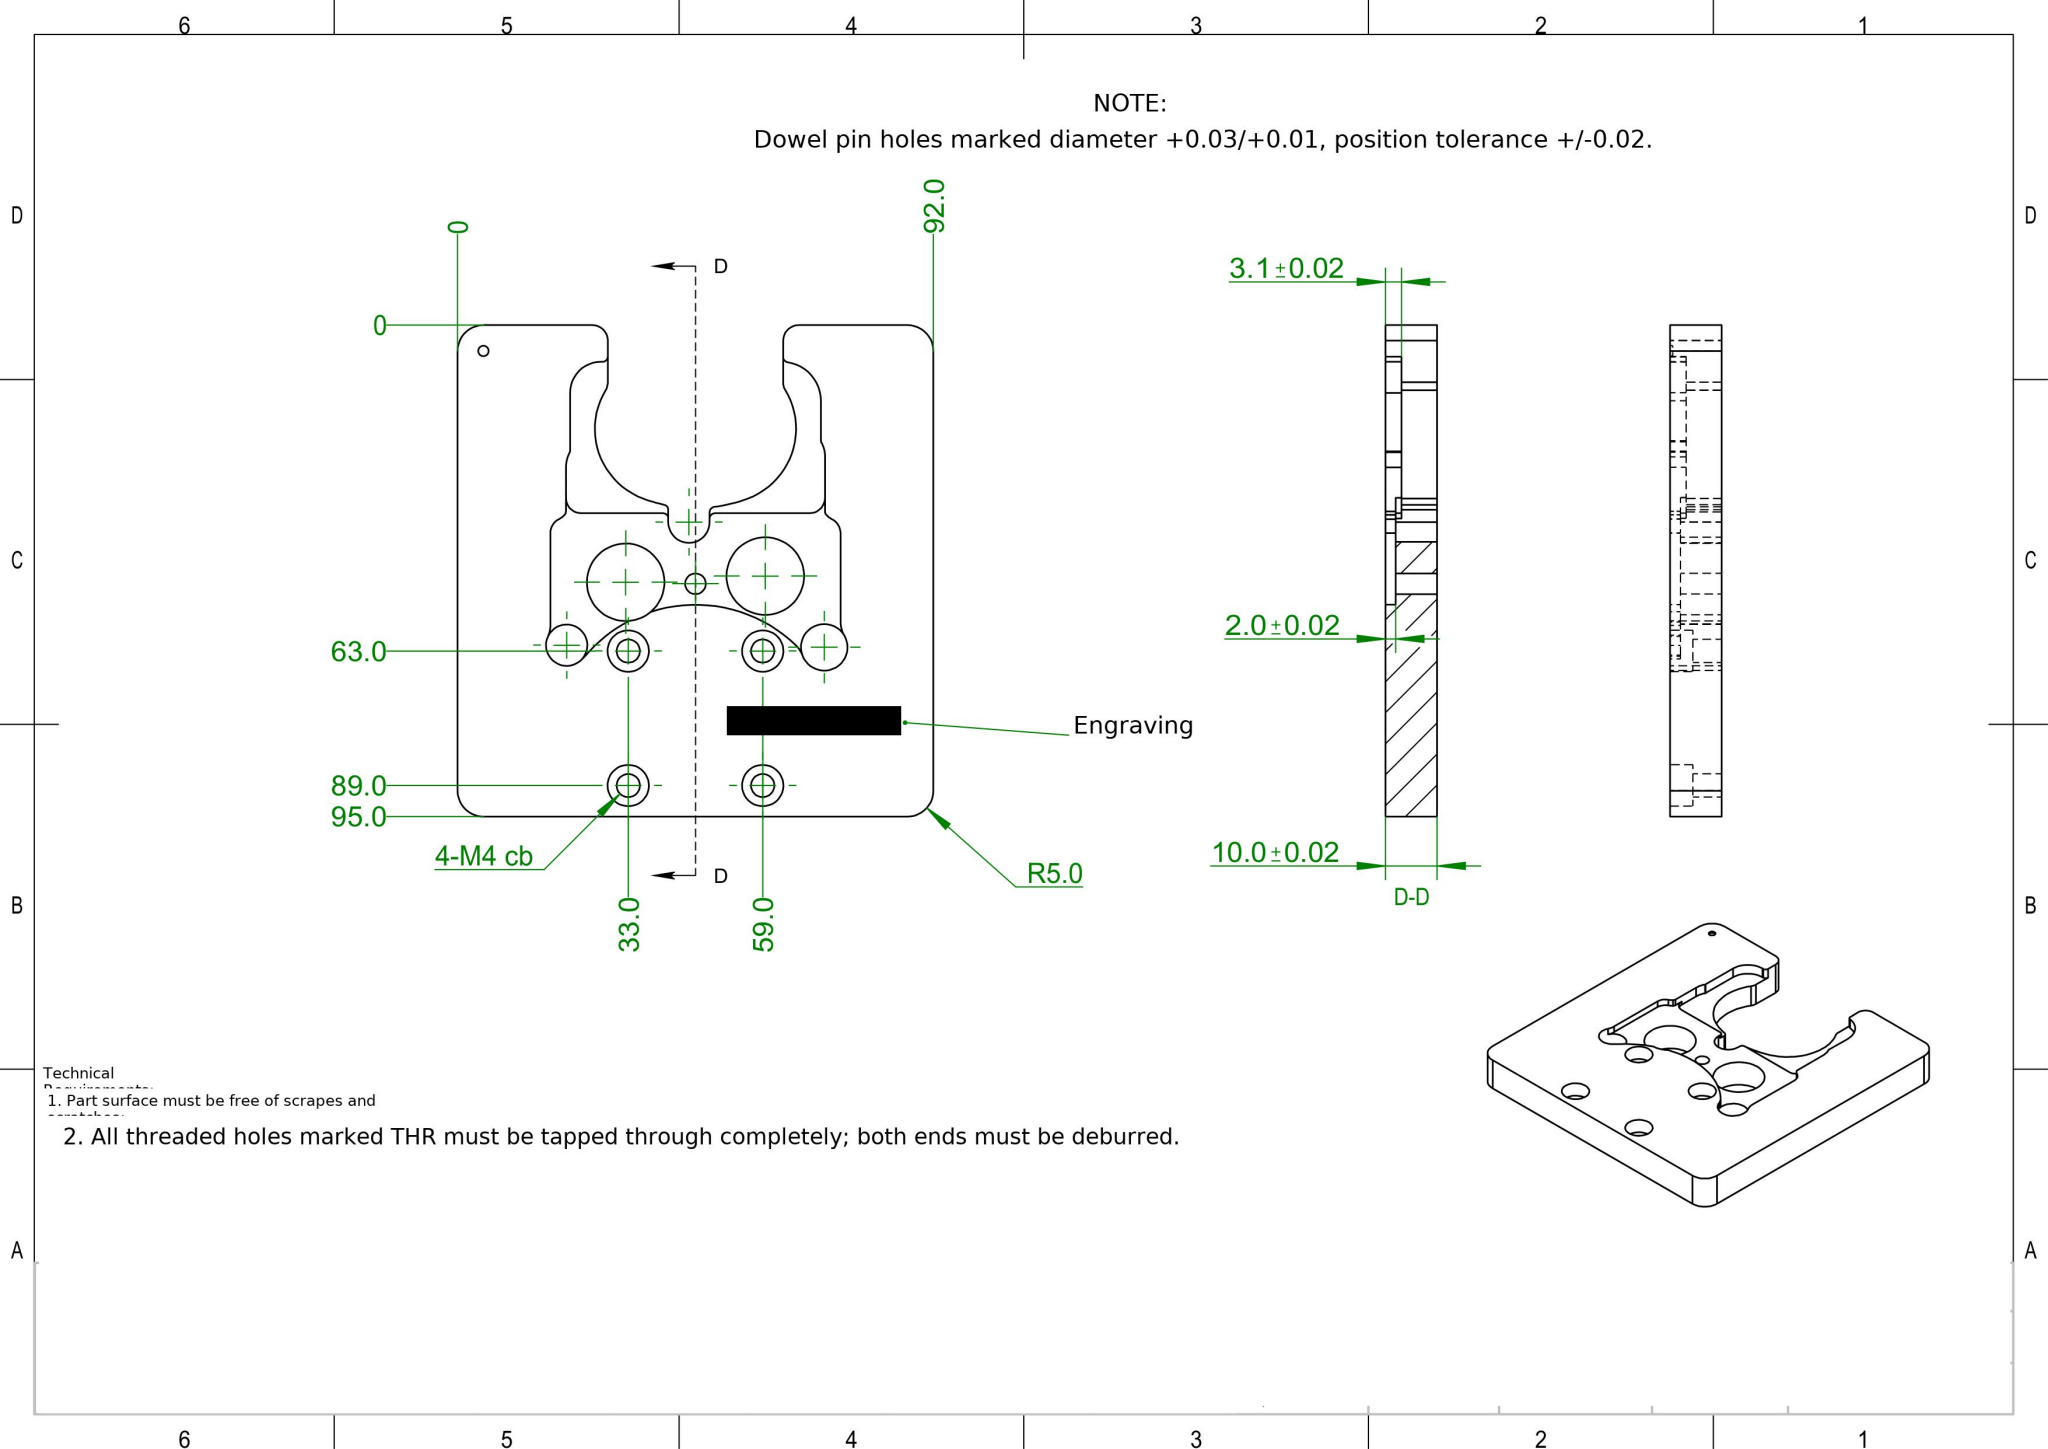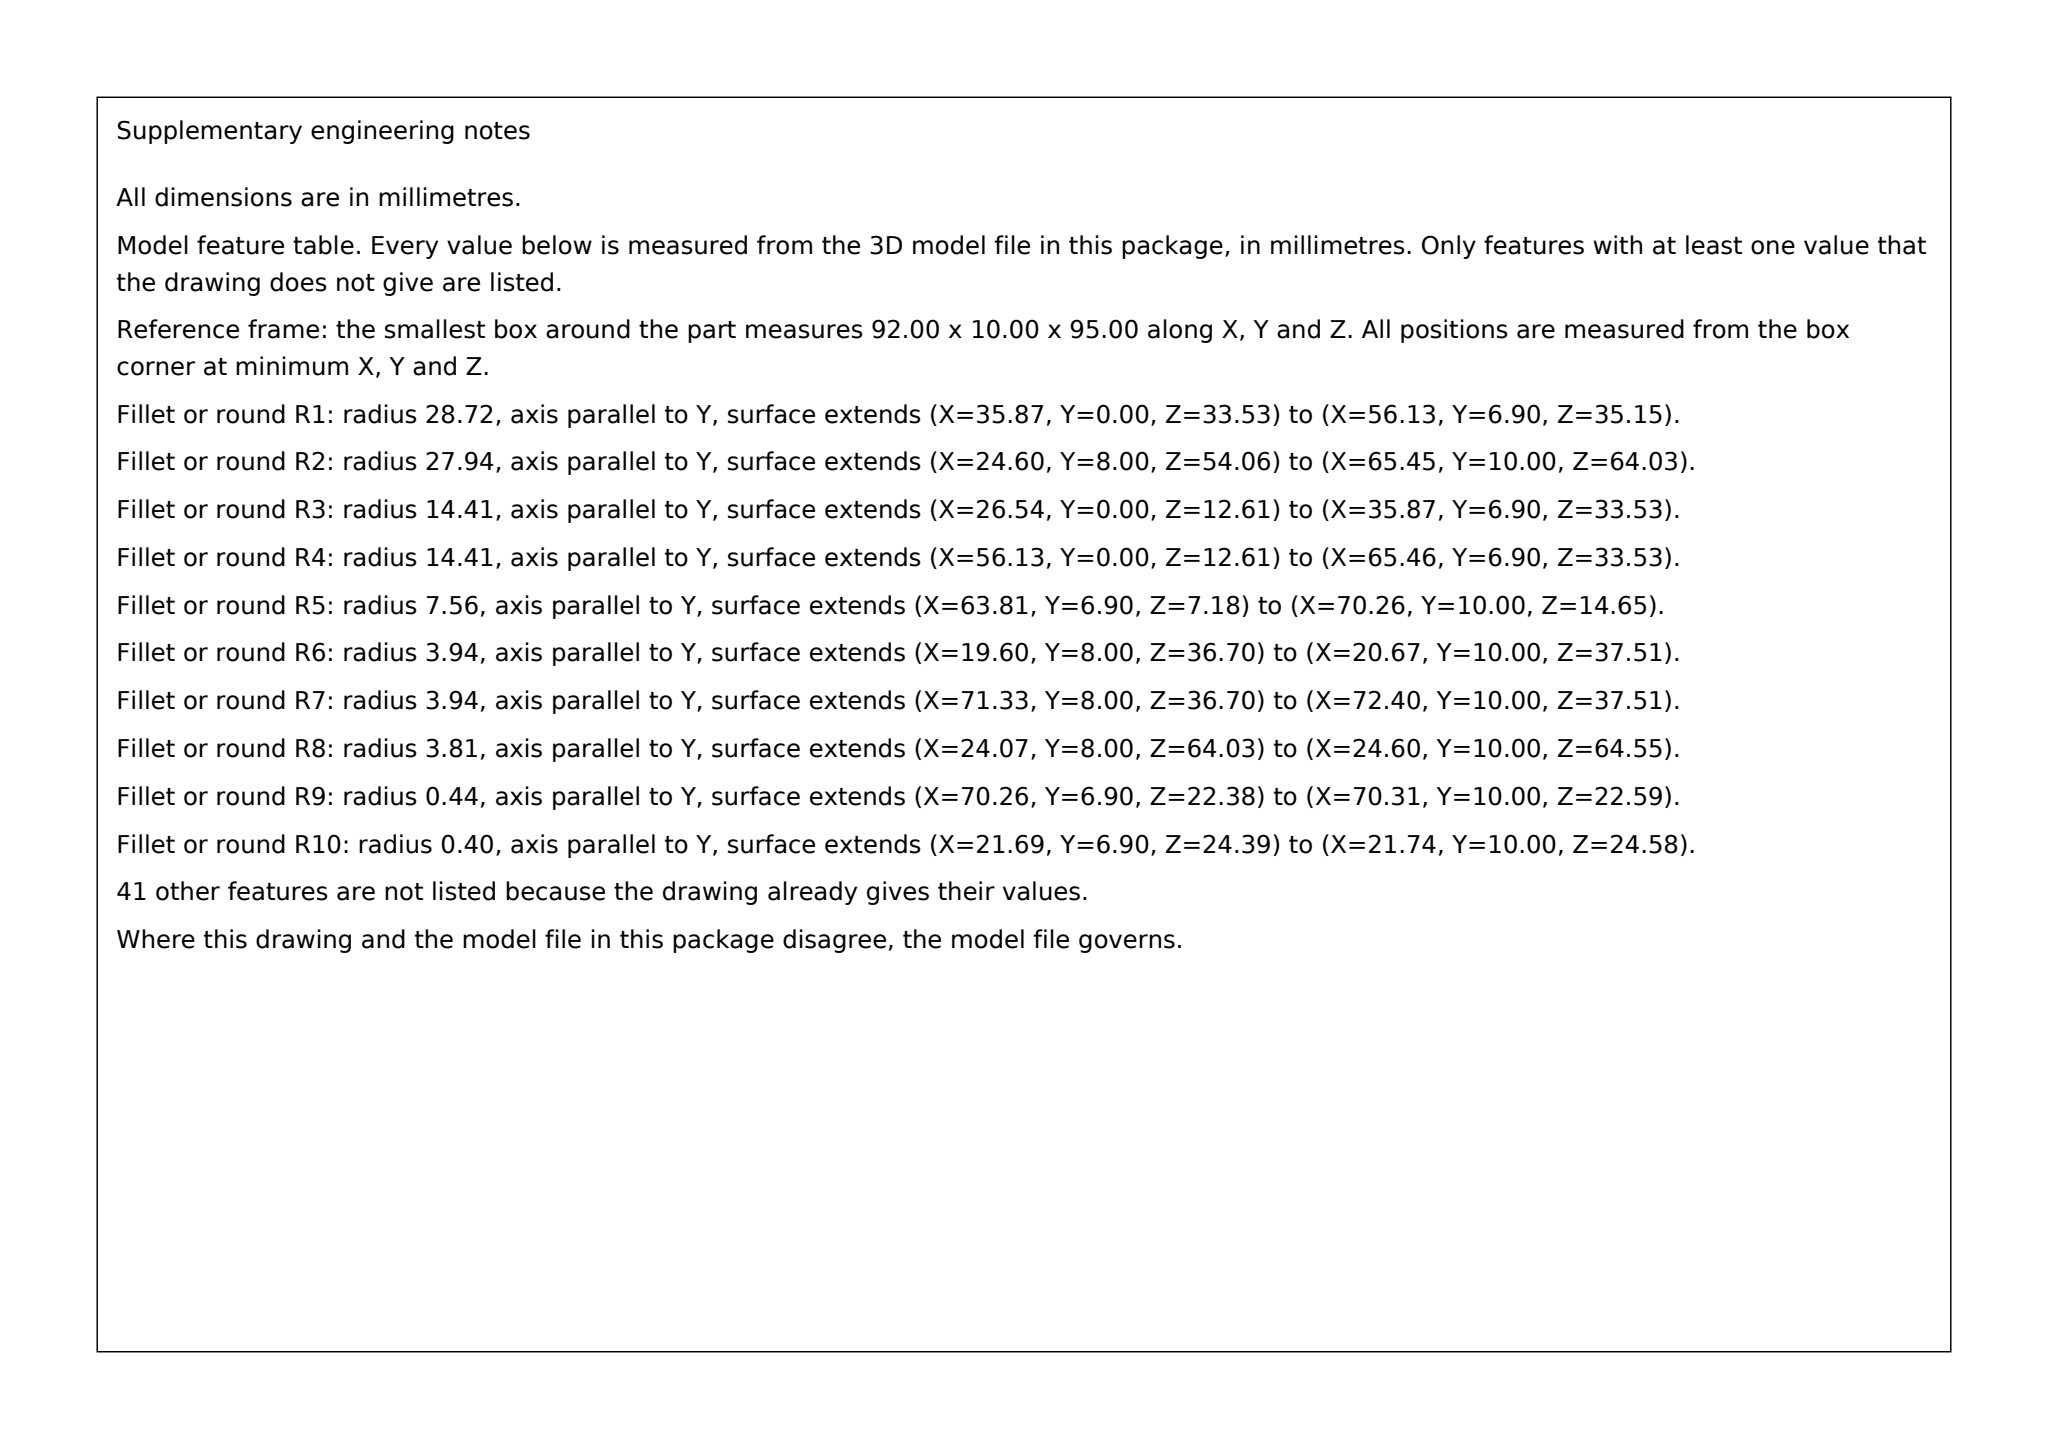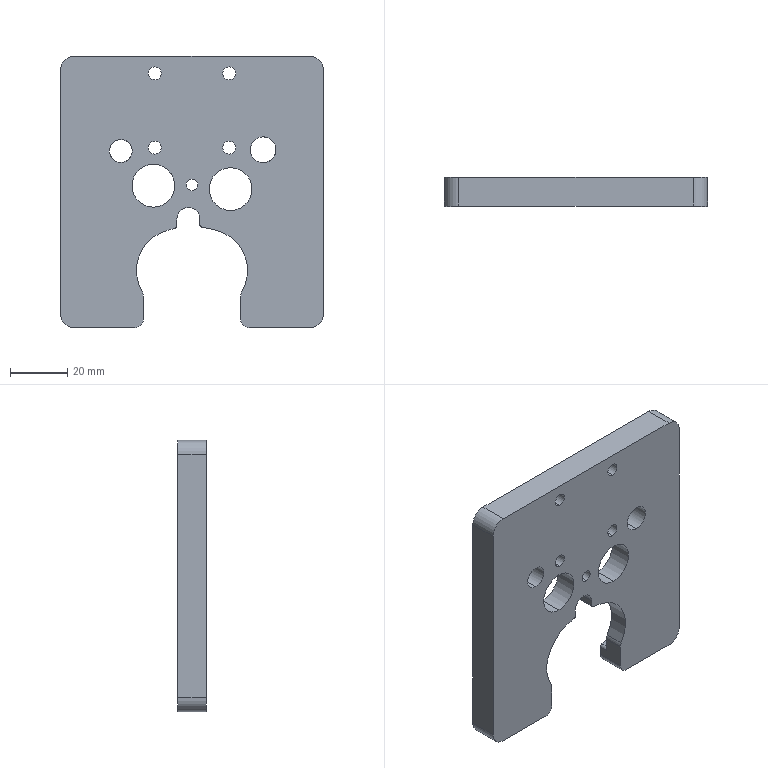Part | SolidWorks | mm | 1 solid | 96 faces | box 92 x 10 x 95 mm | volume 65780 mm3 | cylinder 68 | plane 28 | commonest cylinder face diameters 8 x12 2 x10 4.5 x8 10 x7 6 x6 15 x4 9 x2 4 x2